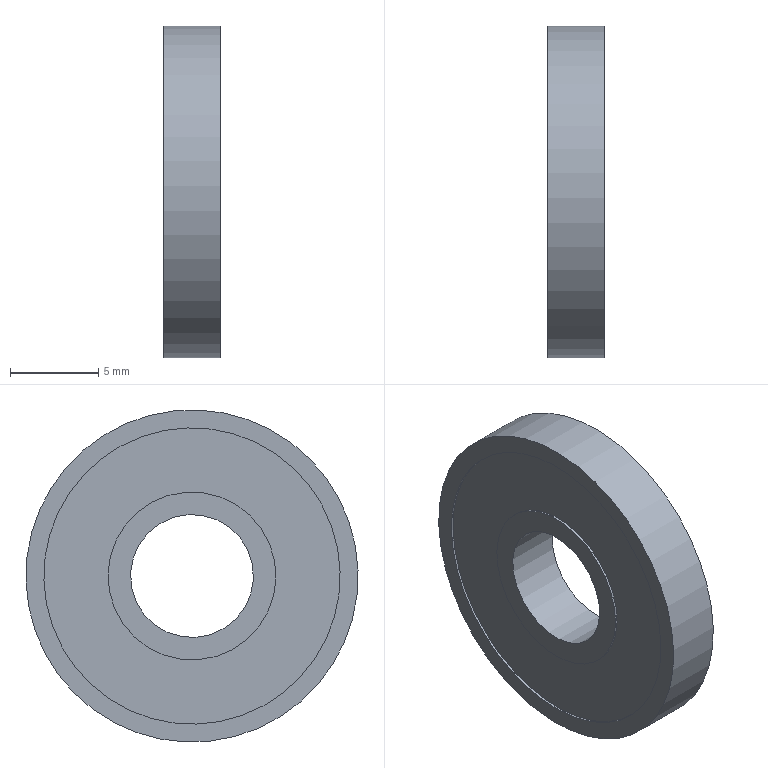Component | NX | BEARINGSMALL | 3 solids | 12 faces | box 3.18 x 18.8 x 18.8 mm | volume 722 mm3 | cylinder 6 | plane 6 | commonest cylinder face diameters 16.764 x2 9.5 x2 18.796 x1 6.96 x1
STEP:
#1=CARTESIAN_POINT('',(0.,0.,0.));
#2=DIRECTION('',(0.,0.,1.));
#3=DIRECTION('',(1.,0.,0.));
#4=AXIS2_PLACEMENT_3D('',#1,#2,#3);
#5=CARTESIAN_POINT('',(-24.892,8.238,-1.547));
#6=VERTEX_POINT('',#5);
#7=CARTESIAN_POINT('',(-24.892,-0.,-0.));
#8=DIRECTION('',(1.,0.,0.));
#9=DIRECTION('',(0.,0.9828,-0.1846));
#10=AXIS2_PLACEMENT_3D('',#7,#8,#9);
#11=CIRCLE('',#10,8.382);
#12=CARTESIAN_POINT('',(-24.892,-0.,-0.));
#13=DIRECTION('',(-1.,0.,0.));
#14=DIRECTION('',(0.,0.1846,0.9828));
#15=AXIS2_PLACEMENT_3D('',#12,#13,#14);
#16=CYLINDRICAL_SURFACE('',#15,8.382);
#17=CARTESIAN_POINT('',(7.854,0.));
#18=DIRECTION('',(-1.,0.));
#19=VECTOR('',#18,1.);
#20=LINE('',#17,#19);
#21=(GEOMETRIC_REPRESENTATION_CONTEXT(2)PARAMETRIC_REPRESENTATION_CONTEXT()REPRESENTATION_CONTEXT('',''));
#22=DEFINITIONAL_REPRESENTATION('',(#20),#21);
#23=PCURVE('',#16,#22);
#24=CARTESIAN_POINT('',(-24.892,-0.,-0.));
#25=DIRECTION('',(1.,0.,0.));
#26=DIRECTION('',(0.,-0.1846,-0.9828));
#27=AXIS2_PLACEMENT_3D('',#24,#25,#26);
#28=PLANE('',#27);
#29=CARTESIAN_POINT('',(0.,0.));
#30=DIRECTION('',(0.,1.));
#31=AXIS2_PLACEMENT_2D('',#29,#30);
#32=CIRCLE('',#31,8.382);
#33=(GEOMETRIC_REPRESENTATION_CONTEXT(2)PARAMETRIC_REPRESENTATION_CONTEXT()REPRESENTATION_CONTEXT('',''));
#34=DEFINITIONAL_REPRESENTATION('',(#32),#33);
#35=PCURVE('',#28,#34);
#36=SURFACE_CURVE('',#11,(#23,#35),.PCURVE_S1.);
#37=EDGE_CURVE('',#6,#6,#36,.T.);
#38=ORIENTED_EDGE('',*,*,#37,.F.);
#39=CARTESIAN_POINT('',(-27.813,8.238,-1.547));
#40=VERTEX_POINT('',#39);
#41=CARTESIAN_POINT('',(-24.892,8.238,-1.547));
#42=CARTESIAN_POINT('',(-27.813,8.238,-1.547));
#43=B_SPLINE_CURVE_WITH_KNOTS('',1,(#41,#42),.UNSPECIFIED.,.F.,.F.,(2,2),(0.,2.921),.PIECEWISE_BEZIER_KNOTS.);
#44=CARTESIAN_POINT('',(7.854,0.));
#45=DIRECTION('',(0.,1.));
#46=VECTOR('',#45,1.);
#47=LINE('',#44,#46);
#48=(GEOMETRIC_REPRESENTATION_CONTEXT(2)PARAMETRIC_REPRESENTATION_CONTEXT()REPRESENTATION_CONTEXT('',''));
#49=DEFINITIONAL_REPRESENTATION('',(#47),#48);
#50=PCURVE('',#16,#49);
#51=CARTESIAN_POINT('',(1.571,0.));
#52=DIRECTION('',(0.,1.));
#53=VECTOR('',#52,1.);
#54=LINE('',#51,#53);
#55=(GEOMETRIC_REPRESENTATION_CONTEXT(2)PARAMETRIC_REPRESENTATION_CONTEXT()REPRESENTATION_CONTEXT('',''));
#56=DEFINITIONAL_REPRESENTATION('',(#54),#55);
#57=PCURVE('',#16,#56);
#58=SEAM_CURVE('',#43,(#50,#57),.PCURVE_S1.);
#59=EDGE_CURVE('',#6,#40,#58,.T.);
#60=ORIENTED_EDGE('',*,*,#59,.T.);
#61=CARTESIAN_POINT('',(-27.813,-0.,-0.));
#62=DIRECTION('',(1.,0.,0.));
#63=DIRECTION('',(0.,0.9828,-0.1846));
#64=AXIS2_PLACEMENT_3D('',#61,#62,#63);
#65=CIRCLE('',#64,8.382);
#66=CARTESIAN_POINT('',(7.854,2.921));
#67=DIRECTION('',(-1.,0.));
#68=VECTOR('',#67,1.);
#69=LINE('',#66,#68);
#70=(GEOMETRIC_REPRESENTATION_CONTEXT(2)PARAMETRIC_REPRESENTATION_CONTEXT()REPRESENTATION_CONTEXT('',''));
#71=DEFINITIONAL_REPRESENTATION('',(#69),#70);
#72=PCURVE('',#16,#71);
#73=CARTESIAN_POINT('',(-27.813,-0.,-0.));
#74=DIRECTION('',(1.,0.,0.));
#75=DIRECTION('',(0.,-0.1846,-0.9828));
#76=AXIS2_PLACEMENT_3D('',#73,#74,#75);
#77=PLANE('',#76);
#78=CARTESIAN_POINT('',(0.,0.));
#79=DIRECTION('',(0.,1.));
#80=AXIS2_PLACEMENT_2D('',#78,#79);
#81=CIRCLE('',#80,8.382);
#82=(GEOMETRIC_REPRESENTATION_CONTEXT(2)PARAMETRIC_REPRESENTATION_CONTEXT()REPRESENTATION_CONTEXT('',''));
#83=DEFINITIONAL_REPRESENTATION('',(#81),#82);
#84=PCURVE('',#77,#83);
#85=SURFACE_CURVE('',#65,(#72,#84),.PCURVE_S1.);
#86=EDGE_CURVE('',#40,#40,#85,.T.);
#87=ORIENTED_EDGE('',*,*,#86,.T.);
#88=ORIENTED_EDGE('',*,*,#59,.F.);
#89=EDGE_LOOP('',(#38,#60,#87,#88));
#90=FACE_BOUND('',#89,.T.);
#91=ADVANCED_FACE('',(#90),#16,.T.);
#92=CARTESIAN_POINT('',(-24.892,4.668,-0.8766));
#93=VERTEX_POINT('',#92);
#94=CARTESIAN_POINT('',(-24.892,-0.,-0.));
#95=DIRECTION('',(1.,0.,0.));
#96=DIRECTION('',(0.,0.9828,-0.1846));
#97=AXIS2_PLACEMENT_3D('',#94,#95,#96);
#98=CIRCLE('',#97,4.75);
#99=CARTESIAN_POINT('',(-24.892,-0.,-0.));
#100=DIRECTION('',(-1.,0.,0.));
#101=DIRECTION('',(0.,0.1846,0.9828));
#102=AXIS2_PLACEMENT_3D('',#99,#100,#101);
#103=CYLINDRICAL_SURFACE('',#102,4.75);
#104=CARTESIAN_POINT('',(7.854,0.));
#105=DIRECTION('',(-1.,0.));
#106=VECTOR('',#105,1.);
#107=LINE('',#104,#106);
#108=(GEOMETRIC_REPRESENTATION_CONTEXT(2)PARAMETRIC_REPRESENTATION_CONTEXT()REPRESENTATION_CONTEXT('',''));
#109=DEFINITIONAL_REPRESENTATION('',(#107),#108);
#110=PCURVE('',#103,#109);
#111=CARTESIAN_POINT('',(0.,0.));
#112=DIRECTION('',(0.,1.));
#113=AXIS2_PLACEMENT_2D('',#111,#112);
#114=CIRCLE('',#113,4.75);
#115=(GEOMETRIC_REPRESENTATION_CONTEXT(2)PARAMETRIC_REPRESENTATION_CONTEXT()REPRESENTATION_CONTEXT('',''));
#116=DEFINITIONAL_REPRESENTATION('',(#114),#115);
#117=PCURVE('',#28,#116);
#118=SURFACE_CURVE('',#98,(#110,#117),.PCURVE_S1.);
#119=EDGE_CURVE('',#93,#93,#118,.T.);
#120=ORIENTED_EDGE('',*,*,#119,.F.);
#121=CARTESIAN_POINT('',(-27.813,4.668,-0.8766));
#122=VERTEX_POINT('',#121);
#123=CARTESIAN_POINT('',(-24.892,4.668,-0.8766));
#124=CARTESIAN_POINT('',(-27.813,4.668,-0.8766));
#125=B_SPLINE_CURVE_WITH_KNOTS('',1,(#123,#124),.UNSPECIFIED.,.F.,.F.,(2,2),(0.,2.921),.PIECEWISE_BEZIER_KNOTS.);
#126=CARTESIAN_POINT('',(7.854,0.));
#127=DIRECTION('',(0.,1.));
#128=VECTOR('',#127,1.);
#129=LINE('',#126,#128);
#130=(GEOMETRIC_REPRESENTATION_CONTEXT(2)PARAMETRIC_REPRESENTATION_CONTEXT()REPRESENTATION_CONTEXT('',''));
#131=DEFINITIONAL_REPRESENTATION('',(#129),#130);
#132=PCURVE('',#103,#131);
#133=CARTESIAN_POINT('',(1.571,0.));
#134=DIRECTION('',(0.,1.));
#135=VECTOR('',#134,1.);
#136=LINE('',#133,#135);
#137=(GEOMETRIC_REPRESENTATION_CONTEXT(2)PARAMETRIC_REPRESENTATION_CONTEXT()REPRESENTATION_CONTEXT('',''));
#138=DEFINITIONAL_REPRESENTATION('',(#136),#137);
#139=PCURVE('',#103,#138);
#140=SEAM_CURVE('',#125,(#132,#139),.PCURVE_S1.);
#141=EDGE_CURVE('',#93,#122,#140,.T.);
#142=ORIENTED_EDGE('',*,*,#141,.T.);
#143=CARTESIAN_POINT('',(-27.813,-0.,-0.));
#144=DIRECTION('',(1.,0.,0.));
#145=DIRECTION('',(0.,0.9828,-0.1846));
#146=AXIS2_PLACEMENT_3D('',#143,#144,#145);
#147=CIRCLE('',#146,4.75);
#148=CARTESIAN_POINT('',(7.854,2.921));
#149=DIRECTION('',(-1.,0.));
#150=VECTOR('',#149,1.);
#151=LINE('',#148,#150);
#152=(GEOMETRIC_REPRESENTATION_CONTEXT(2)PARAMETRIC_REPRESENTATION_CONTEXT()REPRESENTATION_CONTEXT('',''));
#153=DEFINITIONAL_REPRESENTATION('',(#151),#152);
#154=PCURVE('',#103,#153);
#155=CARTESIAN_POINT('',(0.,0.));
#156=DIRECTION('',(0.,1.));
#157=AXIS2_PLACEMENT_2D('',#155,#156);
#158=CIRCLE('',#157,4.75);
#159=(GEOMETRIC_REPRESENTATION_CONTEXT(2)PARAMETRIC_REPRESENTATION_CONTEXT()REPRESENTATION_CONTEXT('',''));
#160=DEFINITIONAL_REPRESENTATION('',(#158),#159);
#161=PCURVE('',#77,#160);
#162=SURFACE_CURVE('',#147,(#154,#161),.PCURVE_S1.);
#163=EDGE_CURVE('',#122,#122,#162,.T.);
#164=ORIENTED_EDGE('',*,*,#163,.T.);
#165=ORIENTED_EDGE('',*,*,#141,.F.);
#166=EDGE_LOOP('',(#120,#142,#164,#165));
#167=FACE_BOUND('',#166,.F.);
#168=ADVANCED_FACE('',(#167),#103,.F.);
#169=ORIENTED_EDGE('',*,*,#37,.T.);
#170=EDGE_LOOP('',(#169));
#171=FACE_BOUND('',#170,.T.);
#172=ORIENTED_EDGE('',*,*,#119,.F.);
#173=EDGE_LOOP('',(#172));
#174=FACE_BOUND('',#173,.T.);
#175=ADVANCED_FACE('',(#171,#174),#28,.T.);
#176=ORIENTED_EDGE('',*,*,#86,.F.);
#177=EDGE_LOOP('',(#176));
#178=FACE_BOUND('',#177,.T.);
#179=ORIENTED_EDGE('',*,*,#163,.T.);
#180=EDGE_LOOP('',(#179));
#181=FACE_BOUND('',#180,.T.);
#182=ADVANCED_FACE('',(#178,#181),#77,.F.);
#183=CLOSED_SHELL('',(#91,#168,#175,#182));
#184=MANIFOLD_SOLID_BREP('',#183);
#185=(LENGTH_UNIT()NAMED_UNIT(*)SI_UNIT(.MILLI.,.METRE.));
#186=UNCERTAINTY_MEASURE_WITH_UNIT(LENGTH_MEASURE(0.00001),#185,'','');
#187=(NAMED_UNIT(*)PLANE_ANGLE_UNIT()SI_UNIT($,.RADIAN.));
#188=(NAMED_UNIT(*)SI_UNIT($,.STERADIAN.)SOLID_ANGLE_UNIT());
#189=(GEOMETRIC_REPRESENTATION_CONTEXT(3)GLOBAL_UNCERTAINTY_ASSIGNED_CONTEXT((#186))GLOBAL_UNIT_ASSIGNED_CONTEXT((#185,#187,#188))REPRESENTATION_CONTEXT('',''));
#190=ADVANCED_BREP_SHAPE_REPRESENTATION('',(#4,#184),#189);
#191=CARTESIAN_POINT('',(0.,0.,0.));
#192=DIRECTION('',(0.,0.,1.));
#193=DIRECTION('',(1.,0.,0.));
#194=AXIS2_PLACEMENT_3D('',#191,#192,#193);
#195=CARTESIAN_POINT('',(0.,0.,0.));
#196=DIRECTION('',(0.,0.,1.));
#197=DIRECTION('',(1.,0.,0.));
#198=AXIS2_PLACEMENT_3D('',#195,#196,#197);
#199=CARTESIAN_POINT('',(0.,0.,0.));
#200=DIRECTION('',(0.,0.,1.));
#201=DIRECTION('',(1.,0.,0.));
#202=AXIS2_PLACEMENT_3D('',#199,#200,#201);
#203=(LENGTH_UNIT()NAMED_UNIT(*)SI_UNIT(.MILLI.,.METRE.));
#204=UNCERTAINTY_MEASURE_WITH_UNIT(LENGTH_MEASURE(0.00001),#203,'','');
#205=(NAMED_UNIT(*)PLANE_ANGLE_UNIT()SI_UNIT($,.RADIAN.));
#206=(NAMED_UNIT(*)SI_UNIT($,.STERADIAN.)SOLID_ANGLE_UNIT());
#207=(GEOMETRIC_REPRESENTATION_CONTEXT(3)GLOBAL_UNCERTAINTY_ASSIGNED_CONTEXT((#204))GLOBAL_UNIT_ASSIGNED_CONTEXT((#203,#205,#206))REPRESENTATION_CONTEXT('',''));
#208=SHAPE_REPRESENTATION('',(#4,#194,#198,#202),#207);
#209=ITEM_DEFINED_TRANSFORMATION('','',#4,#194);
#210=(REPRESENTATION_RELATIONSHIP('','',#190,#208)REPRESENTATION_RELATIONSHIP_WITH_TRANSFORMATION(#209)SHAPE_REPRESENTATION_RELATIONSHIP());
#211=CARTESIAN_POINT('',(-24.765,9.237,-1.734));
#212=VERTEX_POINT('',#211);
#213=CARTESIAN_POINT('',(-24.765,-0.,-0.));
#214=DIRECTION('',(1.,0.,0.));
#215=DIRECTION('',(0.,0.9828,-0.1846));
#216=AXIS2_PLACEMENT_3D('',#213,#214,#215);
#217=CIRCLE('',#216,9.398);
#218=CARTESIAN_POINT('',(-24.765,-0.,-0.));
#219=DIRECTION('',(-1.,0.,0.));
#220=DIRECTION('',(0.,0.1846,0.9828));
#221=AXIS2_PLACEMENT_3D('',#218,#219,#220);
#222=CYLINDRICAL_SURFACE('',#221,9.398);
#223=CARTESIAN_POINT('',(7.854,0.));
#224=DIRECTION('',(-1.,0.));
#225=VECTOR('',#224,1.);
#226=LINE('',#223,#225);
#227=(GEOMETRIC_REPRESENTATION_CONTEXT(2)PARAMETRIC_REPRESENTATION_CONTEXT()REPRESENTATION_CONTEXT('',''));
#228=DEFINITIONAL_REPRESENTATION('',(#226),#227);
#229=PCURVE('',#222,#228);
#230=CARTESIAN_POINT('',(-24.765,-0.,-0.));
#231=DIRECTION('',(1.,0.,0.));
#232=DIRECTION('',(0.,-0.1846,-0.9828));
#233=AXIS2_PLACEMENT_3D('',#230,#231,#232);
#234=PLANE('',#233);
#235=CARTESIAN_POINT('',(0.,0.));
#236=DIRECTION('',(0.,1.));
#237=AXIS2_PLACEMENT_2D('',#235,#236);
#238=CIRCLE('',#237,9.398);
#239=(GEOMETRIC_REPRESENTATION_CONTEXT(2)PARAMETRIC_REPRESENTATION_CONTEXT()REPRESENTATION_CONTEXT('',''));
#240=DEFINITIONAL_REPRESENTATION('',(#238),#239);
#241=PCURVE('',#234,#240);
#242=SURFACE_CURVE('',#217,(#229,#241),.PCURVE_S1.);
#243=EDGE_CURVE('',#212,#212,#242,.T.);
#244=ORIENTED_EDGE('',*,*,#243,.F.);
#245=CARTESIAN_POINT('',(-27.94,9.237,-1.734));
#246=VERTEX_POINT('',#245);
#247=CARTESIAN_POINT('',(-24.765,9.237,-1.734));
#248=CARTESIAN_POINT('',(-27.94,9.237,-1.734));
#249=B_SPLINE_CURVE_WITH_KNOTS('',1,(#247,#248),.UNSPECIFIED.,.F.,.F.,(2,2),(0.,3.175),.PIECEWISE_BEZIER_KNOTS.);
#250=CARTESIAN_POINT('',(7.854,0.));
#251=DIRECTION('',(0.,1.));
#252=VECTOR('',#251,1.);
#253=LINE('',#250,#252);
#254=(GEOMETRIC_REPRESENTATION_CONTEXT(2)PARAMETRIC_REPRESENTATION_CONTEXT()REPRESENTATION_CONTEXT('',''));
#255=DEFINITIONAL_REPRESENTATION('',(#253),#254);
#256=PCURVE('',#222,#255);
#257=CARTESIAN_POINT('',(1.571,0.));
#258=DIRECTION('',(0.,1.));
#259=VECTOR('',#258,1.);
#260=LINE('',#257,#259);
#261=(GEOMETRIC_REPRESENTATION_CONTEXT(2)PARAMETRIC_REPRESENTATION_CONTEXT()REPRESENTATION_CONTEXT('',''));
#262=DEFINITIONAL_REPRESENTATION('',(#260),#261);
#263=PCURVE('',#222,#262);
#264=SEAM_CURVE('',#249,(#256,#263),.PCURVE_S1.);
#265=EDGE_CURVE('',#212,#246,#264,.T.);
#266=ORIENTED_EDGE('',*,*,#265,.T.);
#267=CARTESIAN_POINT('',(-27.94,-0.,-0.));
#268=DIRECTION('',(1.,0.,0.));
#269=DIRECTION('',(0.,0.9828,-0.1846));
#270=AXIS2_PLACEMENT_3D('',#267,#268,#269);
#271=CIRCLE('',#270,9.398);
#272=CARTESIAN_POINT('',(7.854,3.175));
#273=DIRECTION('',(-1.,0.));
#274=VECTOR('',#273,1.);
#275=LINE('',#272,#274);
#276=(GEOMETRIC_REPRESENTATION_CONTEXT(2)PARAMETRIC_REPRESENTATION_CONTEXT()REPRESENTATION_CONTEXT('',''));
#277=DEFINITIONAL_REPRESENTATION('',(#275),#276);
#278=PCURVE('',#222,#277);
#279=CARTESIAN_POINT('',(-27.94,-0.,-0.));
#280=DIRECTION('',(1.,0.,0.));
#281=DIRECTION('',(0.,-0.1846,-0.9828));
#282=AXIS2_PLACEMENT_3D('',#279,#280,#281);
#283=PLANE('',#282);
#284=CARTESIAN_POINT('',(0.,0.));
#285=DIRECTION('',(0.,1.));
#286=AXIS2_PLACEMENT_2D('',#284,#285);
#287=CIRCLE('',#286,9.398);
#288=(GEOMETRIC_REPRESENTATION_CONTEXT(2)PARAMETRIC_REPRESENTATION_CONTEXT()REPRESENTATION_CONTEXT('',''));
#289=DEFINITIONAL_REPRESENTATION('',(#287),#288);
#290=PCURVE('',#283,#289);
#291=SURFACE_CURVE('',#271,(#278,#290),.PCURVE_S1.);
#292=EDGE_CURVE('',#246,#246,#291,.T.);
#293=ORIENTED_EDGE('',*,*,#292,.T.);
#294=ORIENTED_EDGE('',*,*,#265,.F.);
#295=EDGE_LOOP('',(#244,#266,#293,#294));
#296=FACE_BOUND('',#295,.T.);
#297=ADVANCED_FACE('',(#296),#222,.T.);
#298=CARTESIAN_POINT('',(-24.765,8.238,-1.547));
#299=VERTEX_POINT('',#298);
#300=CARTESIAN_POINT('',(-24.765,-0.,-0.));
#301=DIRECTION('',(-1.,0.,0.));
#302=DIRECTION('',(0.,0.9828,-0.1846));
#303=AXIS2_PLACEMENT_3D('',#300,#301,#302);
#304=CIRCLE('',#303,8.382);
#305=CARTESIAN_POINT('',(-24.765,-0.,-0.));
#306=DIRECTION('',(-1.,0.,0.));
#307=DIRECTION('',(0.,0.1846,0.9828));
#308=AXIS2_PLACEMENT_3D('',#305,#306,#307);
#309=CYLINDRICAL_SURFACE('',#308,8.382);
#310=CARTESIAN_POINT('',(1.571,0.));
#311=DIRECTION('',(1.,0.));
#312=VECTOR('',#311,1.);
#313=LINE('',#310,#312);
#314=(GEOMETRIC_REPRESENTATION_CONTEXT(2)PARAMETRIC_REPRESENTATION_CONTEXT()REPRESENTATION_CONTEXT('',''));
#315=DEFINITIONAL_REPRESENTATION('',(#313),#314);
#316=PCURVE('',#309,#315);
#317=CARTESIAN_POINT('',(0.,8.382));
#318=CARTESIAN_POINT('',(14.518,8.382));
#319=CARTESIAN_POINT('',(7.259,-4.191));
#320=CARTESIAN_POINT('',(0.,-16.764));
#321=CARTESIAN_POINT('',(-7.259,-4.191));
#322=CARTESIAN_POINT('',(-14.518,8.382));
#323=CARTESIAN_POINT('',(0.,8.382));
#324=(BOUNDED_CURVE()B_SPLINE_CURVE(2,(#317,#318,#319,#320,#321,#322,#323),.UNSPECIFIED.,.T.,.F.)B_SPLINE_CURVE_WITH_KNOTS((1,2,2,2,2,1),(-2.094,0.,2.094,4.189,6.283,8.378),.UNSPECIFIED.)CURVE()GEOMETRIC_REPRESENTATION_ITEM()RATIONAL_B_SPLINE_CURVE((1.,0.5,1.,0.5,1.,0.5,1.))REPRESENTATION_ITEM(''));
#325=(GEOMETRIC_REPRESENTATION_CONTEXT(2)PARAMETRIC_REPRESENTATION_CONTEXT()REPRESENTATION_CONTEXT('',''));
#326=DEFINITIONAL_REPRESENTATION('',(#324),#325);
#327=PCURVE('',#234,#326);
#328=SURFACE_CURVE('',#304,(#316,#327),.PCURVE_S1.);
#329=EDGE_CURVE('',#299,#299,#328,.T.);
#330=ORIENTED_EDGE('',*,*,#329,.T.);
#331=CARTESIAN_POINT('',(-27.94,8.238,-1.547));
#332=VERTEX_POINT('',#331);
#333=CARTESIAN_POINT('',(-24.765,8.238,-1.547));
#334=CARTESIAN_POINT('',(-27.94,8.238,-1.547));
#335=B_SPLINE_CURVE_WITH_KNOTS('',1,(#333,#334),.UNSPECIFIED.,.F.,.F.,(2,2),(0.,3.175),.PIECEWISE_BEZIER_KNOTS.);
#336=CARTESIAN_POINT('',(7.854,0.));
#337=DIRECTION('',(0.,1.));
#338=VECTOR('',#337,1.);
#339=LINE('',#336,#338);
#340=(GEOMETRIC_REPRESENTATION_CONTEXT(2)PARAMETRIC_REPRESENTATION_CONTEXT()REPRESENTATION_CONTEXT('',''));
#341=DEFINITIONAL_REPRESENTATION('',(#339),#340);
#342=PCURVE('',#309,#341);
#343=CARTESIAN_POINT('',(1.571,0.));
#344=DIRECTION('',(0.,1.));
#345=VECTOR('',#344,1.);
#346=LINE('',#343,#345);
#347=(GEOMETRIC_REPRESENTATION_CONTEXT(2)PARAMETRIC_REPRESENTATION_CONTEXT()REPRESENTATION_CONTEXT('',''));
#348=DEFINITIONAL_REPRESENTATION('',(#346),#347);
#349=PCURVE('',#309,#348);
#350=SEAM_CURVE('',#335,(#342,#349),.PCURVE_S1.);
#351=EDGE_CURVE('',#299,#332,#350,.T.);
#352=ORIENTED_EDGE('',*,*,#351,.T.);
#353=CARTESIAN_POINT('',(-27.94,-0.,-0.));
#354=DIRECTION('',(-1.,0.,0.));
#355=DIRECTION('',(0.,0.9828,-0.1846));
#356=AXIS2_PLACEMENT_3D('',#353,#354,#355);
#357=CIRCLE('',#356,8.382);
#358=CARTESIAN_POINT('',(1.571,3.175));
#359=DIRECTION('',(1.,0.));
#360=VECTOR('',#359,1.);
#361=LINE('',#358,#360);
#362=(GEOMETRIC_REPRESENTATION_CONTEXT(2)PARAMETRIC_REPRESENTATION_CONTEXT()REPRESENTATION_CONTEXT('',''));
#363=DEFINITIONAL_REPRESENTATION('',(#361),#362);
#364=PCURVE('',#309,#363);
#365=CARTESIAN_POINT('',(0.,8.382));
#366=CARTESIAN_POINT('',(14.518,8.382));
#367=CARTESIAN_POINT('',(7.259,-4.191));
#368=CARTESIAN_POINT('',(0.,-16.764));
#369=CARTESIAN_POINT('',(-7.259,-4.191));
#370=CARTESIAN_POINT('',(-14.518,8.382));
#371=CARTESIAN_POINT('',(0.,8.382));
#372=(BOUNDED_CURVE()B_SPLINE_CURVE(2,(#365,#366,#367,#368,#369,#370,#371),.UNSPECIFIED.,.T.,.F.)B_SPLINE_CURVE_WITH_KNOTS((1,2,2,2,2,1),(-2.094,0.,2.094,4.189,6.283,8.378),.UNSPECIFIED.)CURVE()GEOMETRIC_REPRESENTATION_ITEM()RATIONAL_B_SPLINE_CURVE((1.,0.5,1.,0.5,1.,0.5,1.))REPRESENTATION_ITEM(''));
#373=(GEOMETRIC_REPRESENTATION_CONTEXT(2)PARAMETRIC_REPRESENTATION_CONTEXT()REPRESENTATION_CONTEXT('',''));
#374=DEFINITIONAL_REPRESENTATION('',(#372),#373);
#375=PCURVE('',#283,#374);
#376=SURFACE_CURVE('',#357,(#364,#375),.PCURVE_S1.);
#377=EDGE_CURVE('',#332,#332,#376,.T.);
#378=ORIENTED_EDGE('',*,*,#377,.F.);
#379=ORIENTED_EDGE('',*,*,#351,.F.);
#380=EDGE_LOOP('',(#330,#352,#378,#379));
#381=FACE_BOUND('',#380,.F.);
#382=ADVANCED_FACE('',(#381),#309,.F.);
#383=ORIENTED_EDGE('',*,*,#243,.T.);
#384=EDGE_LOOP('',(#383));
#385=FACE_BOUND('',#384,.T.);
#386=ORIENTED_EDGE('',*,*,#329,.T.);
#387=EDGE_LOOP('',(#386));
#388=FACE_BOUND('',#387,.T.);
#389=ADVANCED_FACE('',(#385,#388),#234,.T.);
#390=ORIENTED_EDGE('',*,*,#292,.F.);
#391=EDGE_LOOP('',(#390));
#392=FACE_BOUND('',#391,.T.);
#393=ORIENTED_EDGE('',*,*,#377,.F.);
#394=EDGE_LOOP('',(#393));
#395=FACE_BOUND('',#394,.T.);
#396=ADVANCED_FACE('',(#392,#395),#283,.F.);
#397=CLOSED_SHELL('',(#297,#382,#389,#396));
#398=MANIFOLD_SOLID_BREP('',#397);
#399=(LENGTH_UNIT()NAMED_UNIT(*)SI_UNIT(.MILLI.,.METRE.));
#400=UNCERTAINTY_MEASURE_WITH_UNIT(LENGTH_MEASURE(0.00001),#399,'','');
#401=(NAMED_UNIT(*)PLANE_ANGLE_UNIT()SI_UNIT($,.RADIAN.));
#402=(NAMED_UNIT(*)SI_UNIT($,.STERADIAN.)SOLID_ANGLE_UNIT());
#403=(GEOMETRIC_REPRESENTATION_CONTEXT(3)GLOBAL_UNCERTAINTY_ASSIGNED_CONTEXT((#400))GLOBAL_UNIT_ASSIGNED_CONTEXT((#399,#401,#402))REPRESENTATION_CONTEXT('',''));
#404=ADVANCED_BREP_SHAPE_REPRESENTATION('',(#4,#398),#403);
#405=ITEM_DEFINED_TRANSFORMATION('','',#4,#198);
#406=(REPRESENTATION_RELATIONSHIP('','',#404,#208)REPRESENTATION_RELATIONSHIP_WITH_TRANSFORMATION(#405)SHAPE_REPRESENTATION_RELATIONSHIP());
#407=CARTESIAN_POINT('',(-24.765,4.668,-0.8766));
#408=VERTEX_POINT('',#407);
#409=CARTESIAN_POINT('',(-24.765,-0.,-0.));
#410=DIRECTION('',(-1.,0.,0.));
#411=DIRECTION('',(0.,0.9828,-0.1846));
#412=AXIS2_PLACEMENT_3D('',#409,#410,#411);
#413=CIRCLE('',#412,4.75);
#414=CARTESIAN_POINT('',(-24.765,-0.,-0.));
#415=DIRECTION('',(-1.,0.,0.));
#416=DIRECTION('',(0.,0.1846,0.9828));
#417=AXIS2_PLACEMENT_3D('',#414,#415,#416);
#418=CYLINDRICAL_SURFACE('',#417,4.75);
#419=CARTESIAN_POINT('',(1.571,0.));
#420=DIRECTION('',(1.,0.));
#421=VECTOR('',#420,1.);
#422=LINE('',#419,#421);
#423=(GEOMETRIC_REPRESENTATION_CONTEXT(2)PARAMETRIC_REPRESENTATION_CONTEXT()REPRESENTATION_CONTEXT('',''));
#424=DEFINITIONAL_REPRESENTATION('',(#422),#423);
#425=PCURVE('',#418,#424);
#426=CARTESIAN_POINT('',(-24.765,-0.,-0.));
#427=DIRECTION('',(1.,0.,0.));
#428=DIRECTION('',(0.,-0.1846,-0.9828));
#429=AXIS2_PLACEMENT_3D('',#426,#427,#428);
#430=PLANE('',#429);
#431=CARTESIAN_POINT('',(0.,4.75));
#432=CARTESIAN_POINT('',(8.227,4.75));
#433=CARTESIAN_POINT('',(4.113,-2.375));
#434=CARTESIAN_POINT('',(0.,-9.5));
#435=CARTESIAN_POINT('',(-4.113,-2.375));
#436=CARTESIAN_POINT('',(-8.227,4.75));
#437=CARTESIAN_POINT('',(0.,4.75));
#438=(BOUNDED_CURVE()B_SPLINE_CURVE(2,(#431,#432,#433,#434,#435,#436,#437),.UNSPECIFIED.,.T.,.F.)B_SPLINE_CURVE_WITH_KNOTS((1,2,2,2,2,1),(-2.094,0.,2.094,4.189,6.283,8.378),.UNSPECIFIED.)CURVE()GEOMETRIC_REPRESENTATION_ITEM()RATIONAL_B_SPLINE_CURVE((1.,0.5,1.,0.5,1.,0.5,1.))REPRESENTATION_ITEM(''));
#439=(GEOMETRIC_REPRESENTATION_CONTEXT(2)PARAMETRIC_REPRESENTATION_CONTEXT()REPRESENTATION_CONTEXT('',''));
#440=DEFINITIONAL_REPRESENTATION('',(#438),#439);
#441=PCURVE('',#430,#440);
#442=SURFACE_CURVE('',#413,(#425,#441),.PCURVE_S1.);
#443=EDGE_CURVE('',#408,#408,#442,.T.);
#444=ORIENTED_EDGE('',*,*,#443,.T.);
#445=CARTESIAN_POINT('',(-27.94,4.668,-0.8766));
#446=VERTEX_POINT('',#445);
#447=CARTESIAN_POINT('',(-24.765,4.668,-0.8766));
#448=CARTESIAN_POINT('',(-27.94,4.668,-0.8766));
#449=B_SPLINE_CURVE_WITH_KNOTS('',1,(#447,#448),.UNSPECIFIED.,.F.,.F.,(2,2),(0.,3.175),.PIECEWISE_BEZIER_KNOTS.);
#450=CARTESIAN_POINT('',(7.854,0.));
#451=DIRECTION('',(0.,1.));
#452=VECTOR('',#451,1.);
#453=LINE('',#450,#452);
#454=(GEOMETRIC_REPRESENTATION_CONTEXT(2)PARAMETRIC_REPRESENTATION_CONTEXT()REPRESENTATION_CONTEXT('',''));
#455=DEFINITIONAL_REPRESENTATION('',(#453),#454);
#456=PCURVE('',#418,#455);
#457=CARTESIAN_POINT('',(1.571,0.));
#458=DIRECTION('',(0.,1.));
#459=VECTOR('',#458,1.);
#460=LINE('',#457,#459);
#461=(GEOMETRIC_REPRESENTATION_CONTEXT(2)PARAMETRIC_REPRESENTATION_CONTEXT()REPRESENTATION_CONTEXT('',''));
#462=DEFINITIONAL_REPRESENTATION('',(#460),#461);
#463=PCURVE('',#418,#462);
#464=SEAM_CURVE('',#449,(#456,#463),.PCURVE_S1.);
#465=EDGE_CURVE('',#408,#446,#464,.T.);
#466=ORIENTED_EDGE('',*,*,#465,.T.);
#467=CARTESIAN_POINT('',(-27.94,-0.,-0.));
#468=DIRECTION('',(-1.,0.,0.));
#469=DIRECTION('',(0.,0.9828,-0.1846));
#470=AXIS2_PLACEMENT_3D('',#467,#468,#469);
#471=CIRCLE('',#470,4.75);
#472=CARTESIAN_POINT('',(1.571,3.175));
#473=DIRECTION('',(1.,0.));
#474=VECTOR('',#473,1.);
#475=LINE('',#472,#474);
#476=(GEOMETRIC_REPRESENTATION_CONTEXT(2)PARAMETRIC_REPRESENTATION_CONTEXT()REPRESENTATION_CONTEXT('',''));
#477=DEFINITIONAL_REPRESENTATION('',(#475),#476);
#478=PCURVE('',#418,#477);
#479=CARTESIAN_POINT('',(-27.94,-0.,-0.));
#480=DIRECTION('',(1.,0.,0.));
#481=DIRECTION('',(0.,-0.1846,-0.9828));
#482=AXIS2_PLACEMENT_3D('',#479,#480,#481);
#483=PLANE('',#482);
#484=CARTESIAN_POINT('',(0.,4.75));
#485=CARTESIAN_POINT('',(8.227,4.75));
#486=CARTESIAN_POINT('',(4.113,-2.375));
#487=CARTESIAN_POINT('',(0.,-9.5));
#488=CARTESIAN_POINT('',(-4.113,-2.375));
#489=CARTESIAN_POINT('',(-8.227,4.75));
#490=CARTESIAN_POINT('',(0.,4.75));
#491=(BOUNDED_CURVE()B_SPLINE_CURVE(2,(#484,#485,#486,#487,#488,#489,#490),.UNSPECIFIED.,.T.,.F.)B_SPLINE_CURVE_WITH_KNOTS((1,2,2,2,2,1),(-2.094,0.,2.094,4.189,6.283,8.378),.UNSPECIFIED.)CURVE()GEOMETRIC_REPRESENTATION_ITEM()RATIONAL_B_SPLINE_CURVE((1.,0.5,1.,0.5,1.,0.5,1.))REPRESENTATION_ITEM(''));
#492=(GEOMETRIC_REPRESENTATION_CONTEXT(2)PARAMETRIC_REPRESENTATION_CONTEXT()REPRESENTATION_CONTEXT('',''));
#493=DEFINITIONAL_REPRESENTATION('',(#491),#492);
#494=PCURVE('',#483,#493);
#495=SURFACE_CURVE('',#471,(#478,#494),.PCURVE_S1.);
#496=EDGE_CURVE('',#446,#446,#495,.T.);
#497=ORIENTED_EDGE('',*,*,#496,.F.);
#498=ORIENTED_EDGE('',*,*,#465,.F.);
#499=EDGE_LOOP('',(#444,#466,#497,#498));
#500=FACE_BOUND('',#499,.T.);
#501=ADVANCED_FACE('',(#500),#418,.T.);
#502=CARTESIAN_POINT('',(-24.765,3.42,-0.6422));
#503=VERTEX_POINT('',#502);
#504=CARTESIAN_POINT('',(-24.765,-0.,-0.));
#505=DIRECTION('',(1.,0.,0.));
#506=DIRECTION('',(0.,0.9828,-0.1846));
#507=AXIS2_PLACEMENT_3D('',#504,#505,#506);
#508=CIRCLE('',#507,3.48);
#509=CARTESIAN_POINT('',(-24.765,-0.,-0.));
#510=DIRECTION('',(-1.,0.,0.));
#511=DIRECTION('',(0.,0.1846,0.9828));
#512=AXIS2_PLACEMENT_3D('',#509,#510,#511);
#513=CYLINDRICAL_SURFACE('',#512,3.48);
#514=CARTESIAN_POINT('',(7.854,0.));
#515=DIRECTION('',(-1.,0.));
#516=VECTOR('',#515,1.);
#517=LINE('',#514,#516);
#518=(GEOMETRIC_REPRESENTATION_CONTEXT(2)PARAMETRIC_REPRESENTATION_CONTEXT()REPRESENTATION_CONTEXT('',''));
#519=DEFINITIONAL_REPRESENTATION('',(#517),#518);
#520=PCURVE('',#513,#519);
#521=CARTESIAN_POINT('',(0.,0.));
#522=DIRECTION('',(0.,1.));
#523=AXIS2_PLACEMENT_2D('',#521,#522);
#524=CIRCLE('',#523,3.48);
#525=(GEOMETRIC_REPRESENTATION_CONTEXT(2)PARAMETRIC_REPRESENTATION_CONTEXT()REPRESENTATION_CONTEXT('',''));
#526=DEFINITIONAL_REPRESENTATION('',(#524),#525);
#527=PCURVE('',#430,#526);
#528=SURFACE_CURVE('',#508,(#520,#527),.PCURVE_S1.);
#529=EDGE_CURVE('',#503,#503,#528,.T.);
#530=ORIENTED_EDGE('',*,*,#529,.F.);
#531=CARTESIAN_POINT('',(-27.94,3.42,-0.6422));
#532=VERTEX_POINT('',#531);
#533=CARTESIAN_POINT('',(-24.765,3.42,-0.6422));
#534=CARTESIAN_POINT('',(-27.94,3.42,-0.6422));
#535=B_SPLINE_CURVE_WITH_KNOTS('',1,(#533,#534),.UNSPECIFIED.,.F.,.F.,(2,2),(0.,3.175),.PIECEWISE_BEZIER_KNOTS.);
#536=CARTESIAN_POINT('',(7.854,0.));
#537=DIRECTION('',(0.,1.));
#538=VECTOR('',#537,1.);
#539=LINE('',#536,#538);
#540=(GEOMETRIC_REPRESENTATION_CONTEXT(2)PARAMETRIC_REPRESENTATION_CONTEXT()REPRESENTATION_CONTEXT('',''));
#541=DEFINITIONAL_REPRESENTATION('',(#539),#540);
#542=PCURVE('',#513,#541);
#543=CARTESIAN_POINT('',(1.571,0.));
#544=DIRECTION('',(0.,1.));
#545=VECTOR('',#544,1.);
#546=LINE('',#543,#545);
#547=(GEOMETRIC_REPRESENTATION_CONTEXT(2)PARAMETRIC_REPRESENTATION_CONTEXT()REPRESENTATION_CONTEXT('',''));
#548=DEFINITIONAL_REPRESENTATION('',(#546),#547);
#549=PCURVE('',#513,#548);
#550=SEAM_CURVE('',#535,(#542,#549),.PCURVE_S1.);
#551=EDGE_CURVE('',#503,#532,#550,.T.);
#552=ORIENTED_EDGE('',*,*,#551,.T.);
#553=CARTESIAN_POINT('',(-27.94,-0.,-0.));
#554=DIRECTION('',(1.,0.,0.));
#555=DIRECTION('',(0.,0.9828,-0.1846));
#556=AXIS2_PLACEMENT_3D('',#553,#554,#555);
#557=CIRCLE('',#556,3.48);
#558=CARTESIAN_POINT('',(7.854,3.175));
#559=DIRECTION('',(-1.,0.));
#560=VECTOR('',#559,1.);
#561=LINE('',#558,#560);
#562=(GEOMETRIC_REPRESENTATION_CONTEXT(2)PARAMETRIC_REPRESENTATION_CONTEXT()REPRESENTATION_CONTEXT('',''));
#563=DEFINITIONAL_REPRESENTATION('',(#561),#562);
#564=PCURVE('',#513,#563);
#565=CARTESIAN_POINT('',(0.,0.));
#566=DIRECTION('',(0.,1.));
#567=AXIS2_PLACEMENT_2D('',#565,#566);
#568=CIRCLE('',#567,3.48);
#569=(GEOMETRIC_REPRESENTATION_CONTEXT(2)PARAMETRIC_REPRESENTATION_CONTEXT()REPRESENTATION_CONTEXT('',''));
#570=DEFINITIONAL_REPRESENTATION('',(#568),#569);
#571=PCURVE('',#483,#570);
#572=SURFACE_CURVE('',#557,(#564,#571),.PCURVE_S1.);
#573=EDGE_CURVE('',#532,#532,#572,.T.);
#574=ORIENTED_EDGE('',*,*,#573,.T.);
#575=ORIENTED_EDGE('',*,*,#551,.F.);
#576=EDGE_LOOP('',(#530,#552,#574,#575));
#577=FACE_BOUND('',#576,.F.);
#578=ADVANCED_FACE('',(#577),#513,.F.);
#579=ORIENTED_EDGE('',*,*,#443,.F.);
#580=EDGE_LOOP('',(#579));
#581=FACE_BOUND('',#580,.T.);
#582=ORIENTED_EDGE('',*,*,#529,.F.);
#583=EDGE_LOOP('',(#582));
#584=FACE_BOUND('',#583,.T.);
#585=ADVANCED_FACE('',(#581,#584),#430,.T.);
#586=ORIENTED_EDGE('',*,*,#496,.T.);
#587=EDGE_LOOP('',(#586));
#588=FACE_BOUND('',#587,.T.);
#589=ORIENTED_EDGE('',*,*,#573,.T.);
#590=EDGE_LOOP('',(#589));
#591=FACE_BOUND('',#590,.T.);
#592=ADVANCED_FACE('',(#588,#591),#483,.F.);
#593=CLOSED_SHELL('',(#501,#578,#585,#592));
#594=MANIFOLD_SOLID_BREP('',#593);
#595=(LENGTH_UNIT()NAMED_UNIT(*)SI_UNIT(.MILLI.,.METRE.));
#596=UNCERTAINTY_MEASURE_WITH_UNIT(LENGTH_MEASURE(0.00001),#595,'','');
#597=(NAMED_UNIT(*)PLANE_ANGLE_UNIT()SI_UNIT($,.RADIAN.));
#598=(NAMED_UNIT(*)SI_UNIT($,.STERADIAN.)SOLID_ANGLE_UNIT());
#599=(GEOMETRIC_REPRESENTATION_CONTEXT(3)GLOBAL_UNCERTAINTY_ASSIGNED_CONTEXT((#596))GLOBAL_UNIT_ASSIGNED_CONTEXT((#595,#597,#598))REPRESENTATION_CONTEXT('',''));
#600=ADVANCED_BREP_SHAPE_REPRESENTATION('',(#4,#594),#599);
#601=ITEM_DEFINED_TRANSFORMATION('','',#4,#202);
#602=(REPRESENTATION_RELATIONSHIP('','',#600,#208)REPRESENTATION_RELATIONSHIP_WITH_TRANSFORMATION(#601)SHAPE_REPRESENTATION_RELATIONSHIP());